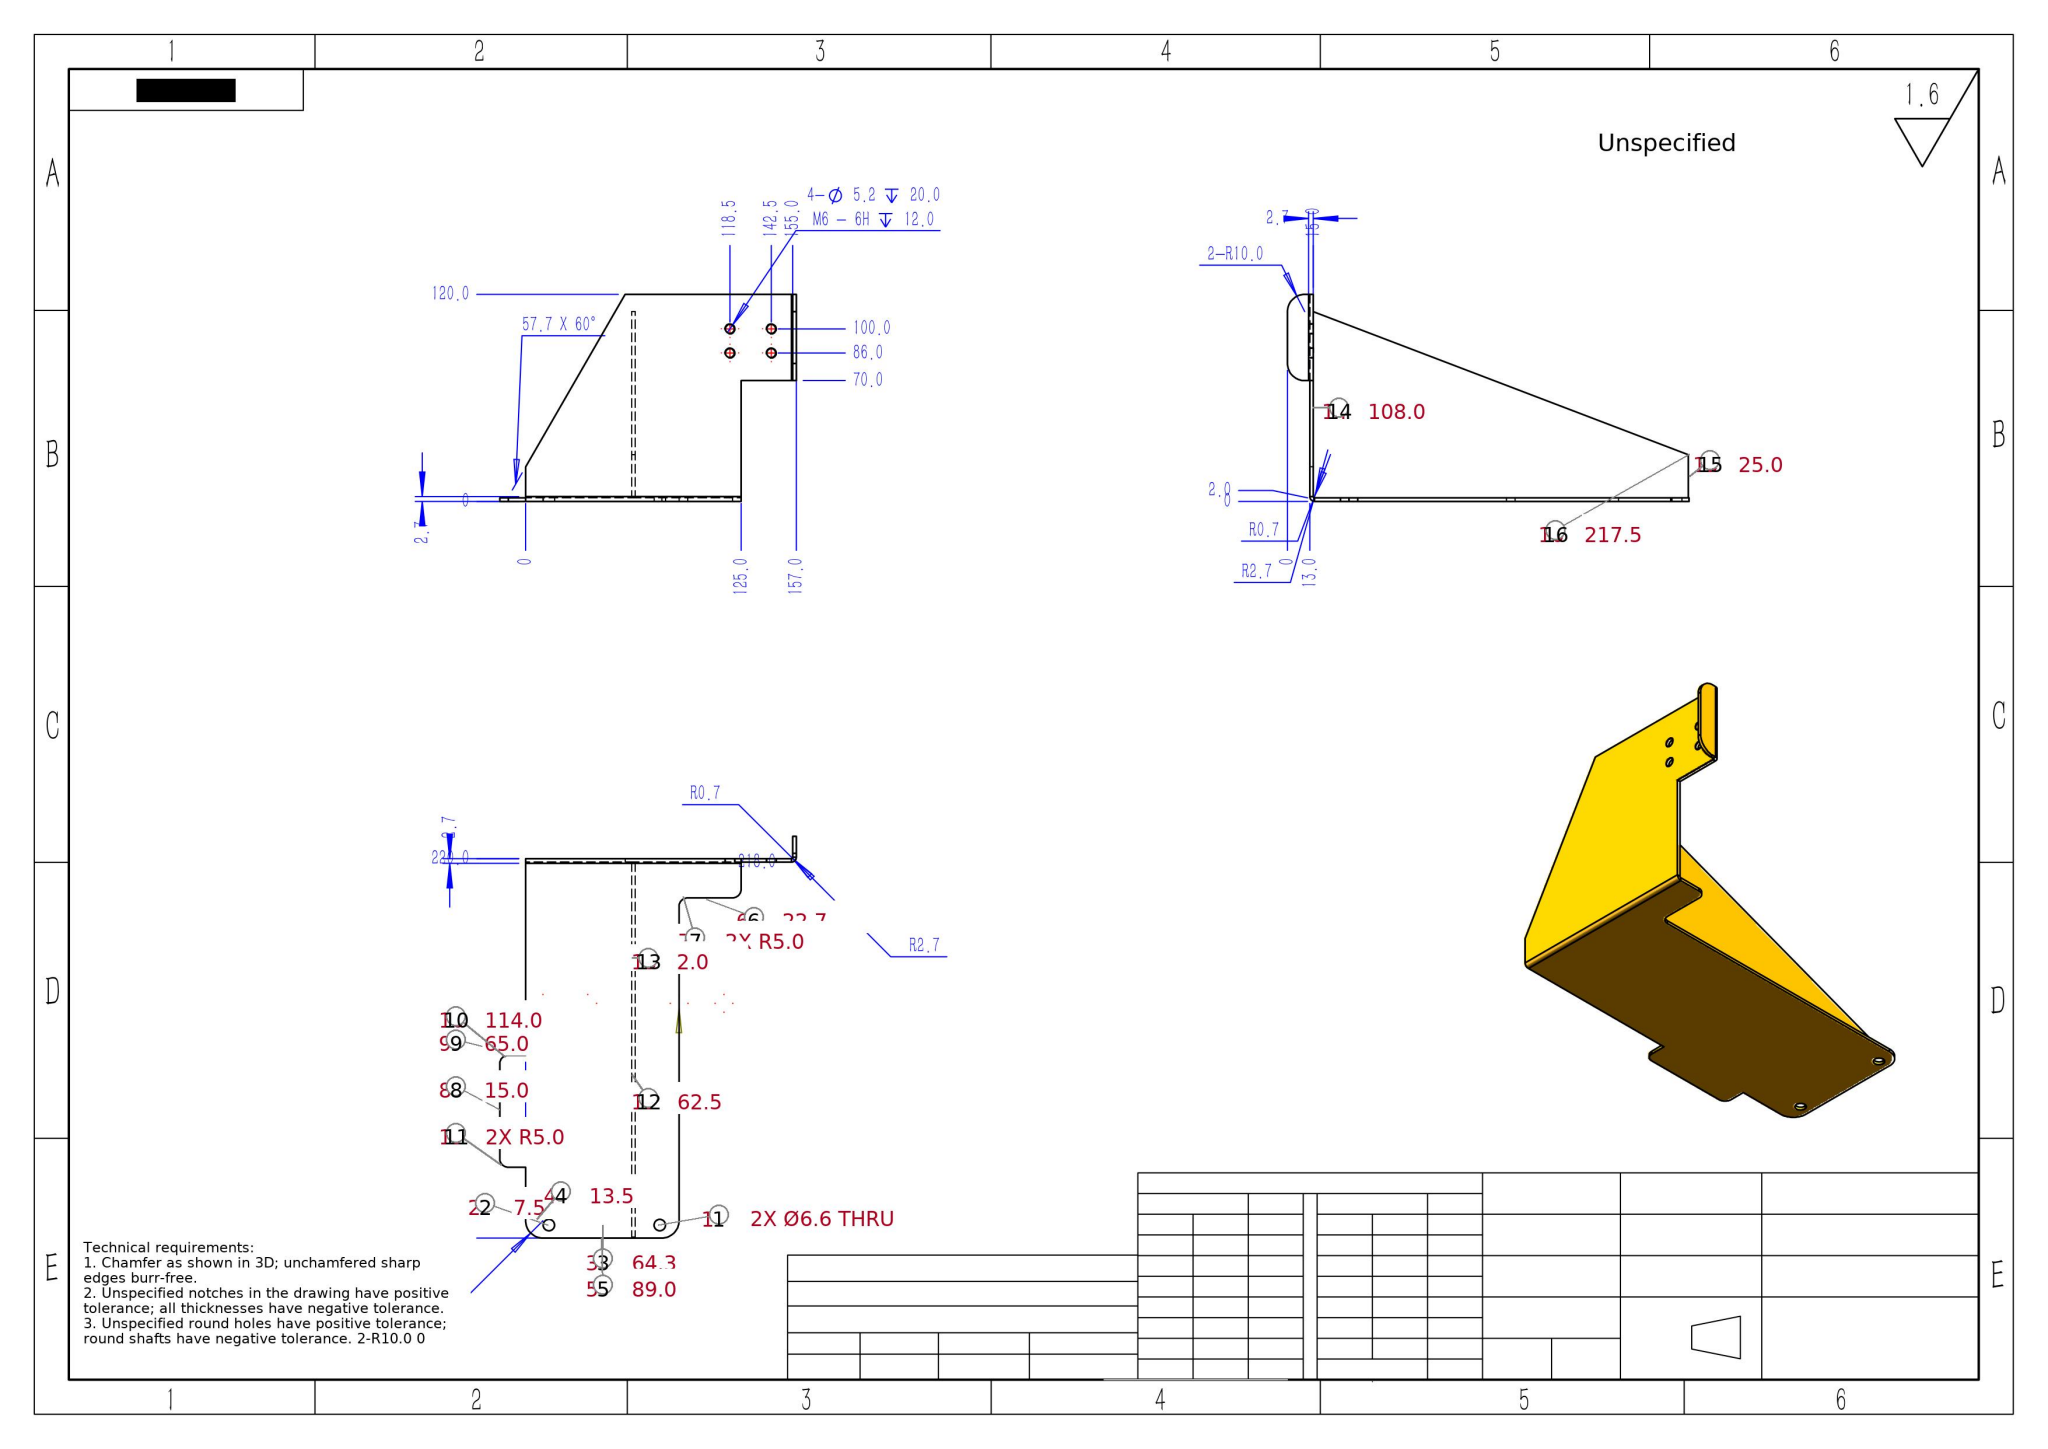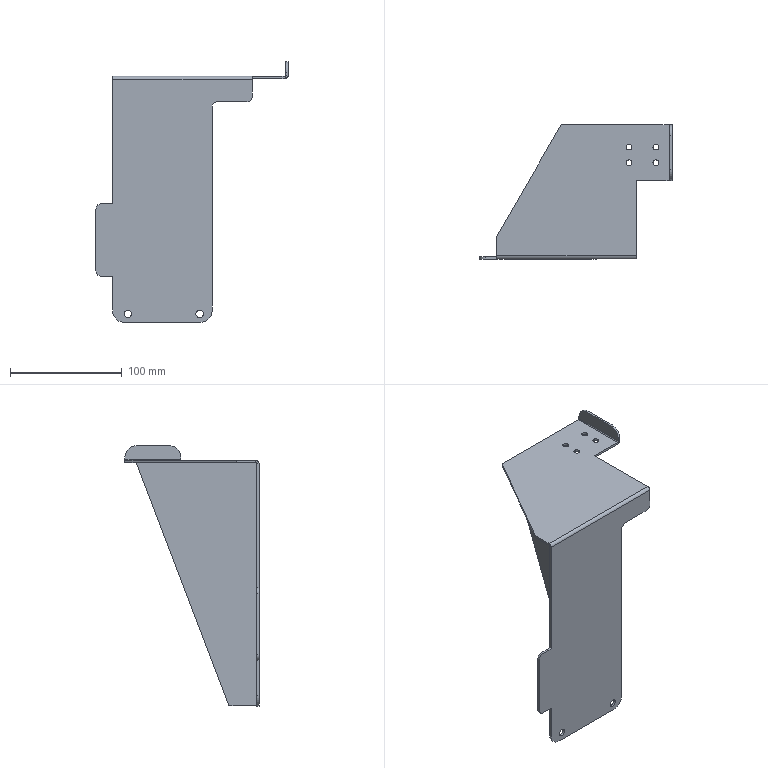Part | SolidWorks | mm | 1 solid | 56 faces | box 172 x 120 x 233 mm | volume 99140 mm3 | plane 31 | cylinder 25 | commonest cylinder face diameters 5.2 x8 6.6 x4 20 x4 10 x4 1.473 x3 5.473 x2